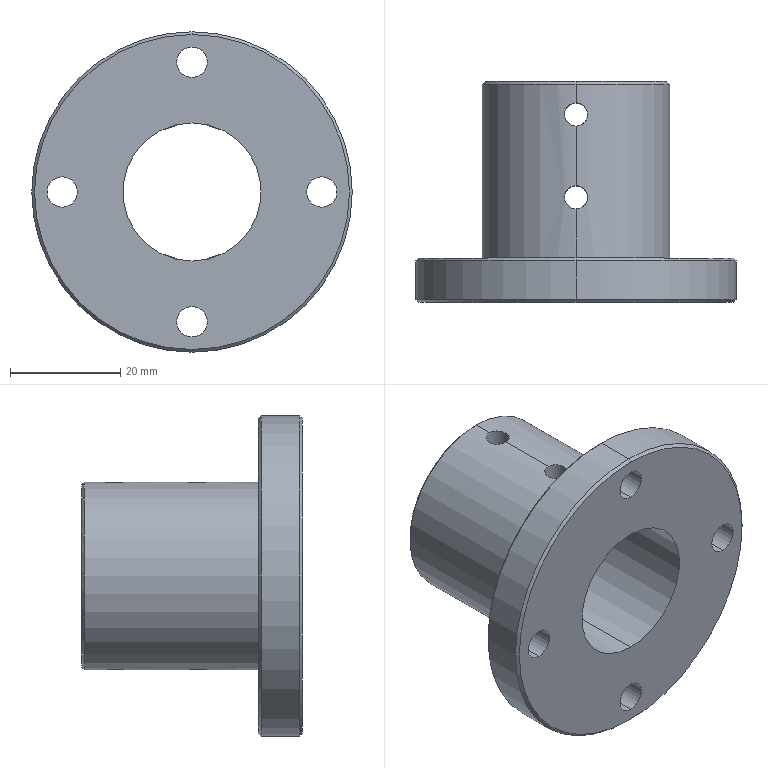Component | SolidWorks | CCDJSSupportColumnFixingRing01-2 | 1 solid | 33 faces | box 58 x 40 x 58 mm | volume 29476 mm3 | cylinder 22 | cone 8 | plane 3 | commonest cylinder face diameters 5.5 x8 4.2 x8 34 x2 58 x2 25 x2 | material 45#
build123d program:
from build123d import *

# Parameters (mm, degrees)
M5_TAPPED_HOLE1_D              = 4.2
F_5_5_5_5_DIAMETER_HOLE1_D     = 5.5
F_5_5_5_5_DIAMETER_HOLE1_DEPTH = 28
F_5_5_5_5_DIAMETER_HOLE1_TIP   = 1.652
CHAMFER1_SIZE                  = 0.5


with BuildPart() as part:
    # Sketch1 → Revolve1 (revolve)
    with BuildSketch(Plane.XY, mode=Mode.PRIVATE) as revolve1_sk:
        Polygon((12.5, 0), (29, 0), (29, 8), (17, 8), (17, 40), (12.5, 40), align=None)
    revolve(revolve1_sk.sketch.rotate(Axis((0, 0, 0), (0, 1, 0)), 90), axis=Axis((0, 0, 0), (0, 1, 0)))

    # M5 Tapped Hole1 (through all)
    with Locations(Plane.XY.offset(17)):
        with Locations((0, 34), (0, 19)):
            Hole(M5_TAPPED_HOLE1_D / 2)

    # 5.5 _5.5_ Diameter Hole1
    with Locations(Plane(origin=(0, 8, 0), x_dir=(1, 0, 0), z_dir=(0, 1, 0))):
        with Locations((0, -23.5), (0, 23.5), (23.5, 0), (-23.5, 0)):
            Hole(F_5_5_5_5_DIAMETER_HOLE1_D / 2, depth=F_5_5_5_5_DIAMETER_HOLE1_DEPTH)
            with Locations((0, 0, -(F_5_5_5_5_DIAMETER_HOLE1_DEPTH + F_5_5_5_5_DIAMETER_HOLE1_TIP / 2))):  # 118° drill point
                Cone(0, F_5_5_5_5_DIAMETER_HOLE1_D / 2, F_5_5_5_5_DIAMETER_HOLE1_TIP, mode=Mode.SUBTRACT)

    # Chamfer1
    chamfer1_edges = [part.edges().sort_by_distance(p)[0] for p in [
        (0, 40, 12.5),
        (0, 40, 17),
        (0, 8, 29),
        (0, 0, 29),
    ]]
    chamfer(chamfer1_edges, length=CHAMFER1_SIZE)


solid = part.part

# Placed as in the assembly
solid = solid.moved(Location((-30, 15, 0), (0, 0, 0)))